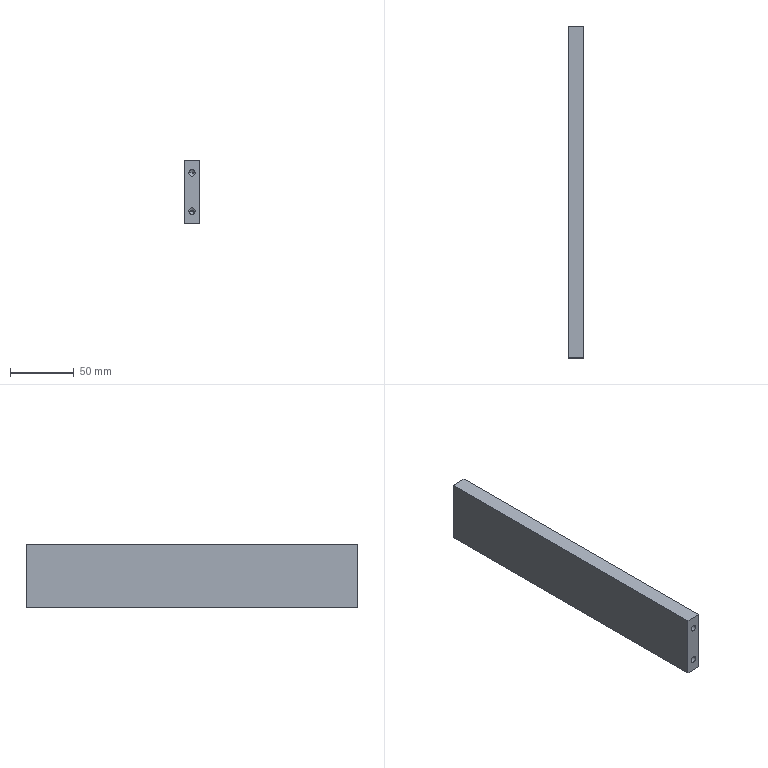Component | SolidWorks | AdjustmentSupportPlate-1 | 1 solid | 22 faces | box 12 x 260 x 50 mm | volume 154783 mm3 | cylinder 8 | cone 8 | plane 6 | commonest cylinder face diameters 5 x8
build123d program:
from build123d import *

# Parameters (mm, degrees)
SKETCH1_W             = 260
SKETCH1_H             = 50
EXTRUDE1_DEPTH        = 12
M6_TAPPED_HOLE1_D     = 5
M6_TAPPED_HOLE1_DEPTH = 15
M6_TAPPED_HOLE1_TIP   = 1.502
M6_TAPPED_HOLE2_D     = 5
M6_TAPPED_HOLE2_DEPTH = 15
M6_TAPPED_HOLE2_TIP   = 1.502


with BuildPart() as part:
    # Sketch1 → Extrude1 (new body)
    with BuildSketch(Plane.XY):
        with Locations((107.997, -15.106)):
            Rectangle(SKETCH1_W, SKETCH1_H)
    extrude(amount=EXTRUDE1_DEPTH)

    # M6 Tapped Hole1
    with Locations(Plane(origin=(237.997, -0.1058, 6), x_dir=(0, 1, 0), z_dir=(1, 0, 0))):
        with Locations((0, 0), (-30, 0)):
            Hole(M6_TAPPED_HOLE1_D / 2, depth=M6_TAPPED_HOLE1_DEPTH)
            with Locations((0, 0, -(M6_TAPPED_HOLE1_DEPTH + M6_TAPPED_HOLE1_TIP / 2))):  # 118° drill point
                Cone(0, M6_TAPPED_HOLE1_D / 2, M6_TAPPED_HOLE1_TIP, mode=Mode.SUBTRACT)

    # M6 Tapped Hole2
    with Locations(Plane(origin=(-22.003, -0.1058, 6), x_dir=(0, -1, 0), z_dir=(-1, 0, 0))):
        with Locations((0, 0), (30, 0)):
            Hole(M6_TAPPED_HOLE2_D / 2, depth=M6_TAPPED_HOLE2_DEPTH)
            with Locations((0, 0, -(M6_TAPPED_HOLE2_DEPTH + M6_TAPPED_HOLE2_TIP / 2))):  # 118° drill point
                Cone(0, M6_TAPPED_HOLE2_D / 2, M6_TAPPED_HOLE2_TIP, mode=Mode.SUBTRACT)


solid = part.part

# Placed as in the assembly
solid = solid.moved(Location((-285.284, 683.98, -65.394), (90, -90, 0)))
STEP:
#1=COLOUR_RGB('',0.7922,0.8196,0.9333);
#2=FILL_AREA_STYLE_COLOUR('',#1);
#3=FILL_AREA_STYLE('',(#2));
#4=SURFACE_STYLE_FILL_AREA(#3);
#5=SURFACE_SIDE_STYLE('',(#4));
#6=SURFACE_STYLE_USAGE(.BOTH.,#5);
#7=PRESENTATION_STYLE_ASSIGNMENT((#6));
#8=CARTESIAN_POINT('',(-11.566,27.204,-3.76));
#9=VERTEX_POINT('',#8);
#10=CARTESIAN_POINT('',(-11.369,27.204,-3.76));
#11=VERTEX_POINT('',#10);
#12=CARTESIAN_POINT('',(-11.468,27.204,-3.76));
#13=DIRECTION('',(-0.,1.,-0.));
#14=DIRECTION('',(1.,0.,-0.));
#15=AXIS2_PLACEMENT_3D('',#12,#13,#14);
#16=CIRCLE('',#15,0.09843);
#17=EDGE_CURVE('',#9,#11,#16,.T.);
#18=ORIENTED_EDGE('',*,*,#17,.F.);
#19=CARTESIAN_POINT('',(-11.566,27.795,-3.76));
#20=VERTEX_POINT('',#19);
#21=CARTESIAN_POINT('',(-11.566,27.795,-3.76));
#22=DIRECTION('',(-0.,1.,-0.));
#23=VECTOR('',#22,39.37);
#24=LINE('',#21,#23);
#25=EDGE_CURVE('',#9,#20,#24,.T.);
#26=ORIENTED_EDGE('',*,*,#25,.T.);
#27=CARTESIAN_POINT('',(-11.369,27.795,-3.76));
#28=VERTEX_POINT('',#27);
#29=CARTESIAN_POINT('',(-11.468,27.795,-3.76));
#30=DIRECTION('',(-0.,1.,-0.));
#31=DIRECTION('',(1.,0.,-0.));
#32=AXIS2_PLACEMENT_3D('',#29,#30,#31);
#33=CIRCLE('',#32,0.09843);
#34=EDGE_CURVE('',#20,#28,#33,.T.);
#35=ORIENTED_EDGE('',*,*,#34,.T.);
#36=CARTESIAN_POINT('',(-11.369,27.795,-3.76));
#37=DIRECTION('',(-0.,1.,-0.));
#38=VECTOR('',#37,39.37);
#39=LINE('',#36,#38);
#40=EDGE_CURVE('',#11,#28,#39,.T.);
#41=ORIENTED_EDGE('',*,*,#40,.F.);
#42=EDGE_LOOP('',(#18,#26,#35,#41));
#43=FACE_OUTER_BOUND('',#42,.T.);
#44=CARTESIAN_POINT('',(-11.468,27.795,-3.76));
#45=DIRECTION('',(-0.,1.,-0.));
#46=DIRECTION('',(1.,0.,-0.));
#47=AXIS2_PLACEMENT_3D('',#44,#45,#46);
#48=CYLINDRICAL_SURFACE('',#47,0.09843);
#49=ADVANCED_FACE('',(#43),#48,.F.);
#50=CARTESIAN_POINT('',(-11.468,27.145,-3.76));
#51=VERTEX_POINT('',#50);
#52=CARTESIAN_POINT('',(-11.369,27.204,-3.76));
#53=DIRECTION('',(0.8572,0.515,-0.));
#54=VECTOR('',#53,39.37);
#55=LINE('',#52,#54);
#56=EDGE_CURVE('',#51,#11,#55,.T.);
#57=ORIENTED_EDGE('',*,*,#56,.F.);
#58=CARTESIAN_POINT('',(-11.566,27.204,-3.76));
#59=DIRECTION('',(-0.8572,0.515,0.));
#60=VECTOR('',#59,39.37);
#61=LINE('',#58,#60);
#62=EDGE_CURVE('',#51,#9,#61,.T.);
#63=ORIENTED_EDGE('',*,*,#62,.T.);
#64=ORIENTED_EDGE('',*,*,#17,.T.);
#65=EDGE_LOOP('',(#57,#63,#64));
#66=FACE_OUTER_BOUND('',#65,.T.);
#67=CARTESIAN_POINT('',(-11.468,27.204,-3.76));
#68=DIRECTION('',(-0.,1.,-0.));
#69=DIRECTION('',(1.,0.,-0.));
#70=AXIS2_PLACEMENT_3D('',#67,#68,#69);
#71=CONICAL_SURFACE('',#70,0.09843,1.03);
#72=ADVANCED_FACE('',(#66),#71,.F.);
#73=CARTESIAN_POINT('',(-11.566,27.204,-2.579));
#74=VERTEX_POINT('',#73);
#75=CARTESIAN_POINT('',(-11.369,27.204,-2.579));
#76=VERTEX_POINT('',#75);
#77=CARTESIAN_POINT('',(-11.468,27.204,-2.579));
#78=DIRECTION('',(-0.,1.,-0.));
#79=DIRECTION('',(1.,0.,-0.));
#80=AXIS2_PLACEMENT_3D('',#77,#78,#79);
#81=CIRCLE('',#80,0.09843);
#82=EDGE_CURVE('',#74,#76,#81,.T.);
#83=ORIENTED_EDGE('',*,*,#82,.F.);
#84=CARTESIAN_POINT('',(-11.566,27.795,-2.579));
#85=VERTEX_POINT('',#84);
#86=CARTESIAN_POINT('',(-11.566,27.795,-2.579));
#87=DIRECTION('',(-0.,1.,-0.));
#88=VECTOR('',#87,39.37);
#89=LINE('',#86,#88);
#90=EDGE_CURVE('',#74,#85,#89,.T.);
#91=ORIENTED_EDGE('',*,*,#90,.T.);
#92=CARTESIAN_POINT('',(-11.369,27.795,-2.579));
#93=VERTEX_POINT('',#92);
#94=CARTESIAN_POINT('',(-11.468,27.795,-2.579));
#95=DIRECTION('',(-0.,1.,-0.));
#96=DIRECTION('',(1.,0.,-0.));
#97=AXIS2_PLACEMENT_3D('',#94,#95,#96);
#98=CIRCLE('',#97,0.09843);
#99=EDGE_CURVE('',#85,#93,#98,.T.);
#100=ORIENTED_EDGE('',*,*,#99,.T.);
#101=CARTESIAN_POINT('',(-11.369,27.795,-2.579));
#102=DIRECTION('',(-0.,1.,-0.));
#103=VECTOR('',#102,39.37);
#104=LINE('',#101,#103);
#105=EDGE_CURVE('',#76,#93,#104,.T.);
#106=ORIENTED_EDGE('',*,*,#105,.F.);
#107=EDGE_LOOP('',(#83,#91,#100,#106));
#108=FACE_OUTER_BOUND('',#107,.T.);
#109=CARTESIAN_POINT('',(-11.468,27.795,-2.579));
#110=DIRECTION('',(-0.,1.,-0.));
#111=DIRECTION('',(1.,0.,-0.));
#112=AXIS2_PLACEMENT_3D('',#109,#110,#111);
#113=CYLINDRICAL_SURFACE('',#112,0.09843);
#114=ADVANCED_FACE('',(#108),#113,.F.);
#115=CARTESIAN_POINT('',(-11.468,27.145,-2.579));
#116=VERTEX_POINT('',#115);
#117=CARTESIAN_POINT('',(-11.369,27.204,-2.579));
#118=DIRECTION('',(0.8572,0.515,-0.));
#119=VECTOR('',#118,39.37);
#120=LINE('',#117,#119);
#121=EDGE_CURVE('',#116,#76,#120,.T.);
#122=ORIENTED_EDGE('',*,*,#121,.F.);
#123=CARTESIAN_POINT('',(-11.566,27.204,-2.579));
#124=DIRECTION('',(-0.8572,0.515,0.));
#125=VECTOR('',#124,39.37);
#126=LINE('',#123,#125);
#127=EDGE_CURVE('',#116,#74,#126,.T.);
#128=ORIENTED_EDGE('',*,*,#127,.T.);
#129=ORIENTED_EDGE('',*,*,#82,.T.);
#130=EDGE_LOOP('',(#122,#128,#129));
#131=FACE_OUTER_BOUND('',#130,.T.);
#132=CARTESIAN_POINT('',(-11.468,27.204,-2.579));
#133=DIRECTION('',(-0.,1.,-0.));
#134=DIRECTION('',(1.,0.,-0.));
#135=AXIS2_PLACEMENT_3D('',#132,#133,#134);
#136=CONICAL_SURFACE('',#135,0.09843,1.03);
#137=ADVANCED_FACE('',(#131),#136,.F.);
#138=CARTESIAN_POINT('',(-11.369,18.149,-3.76));
#139=VERTEX_POINT('',#138);
#140=CARTESIAN_POINT('',(-11.566,18.149,-3.76));
#141=VERTEX_POINT('',#140);
#142=CARTESIAN_POINT('',(-11.468,18.149,-3.76));
#143=DIRECTION('',(0.,-1.,0.));
#144=DIRECTION('',(-1.,0.,0.));
#145=AXIS2_PLACEMENT_3D('',#142,#143,#144);
#146=CIRCLE('',#145,0.09843);
#147=EDGE_CURVE('',#139,#141,#146,.T.);
#148=ORIENTED_EDGE('',*,*,#147,.F.);
#149=CARTESIAN_POINT('',(-11.369,17.558,-3.76));
#150=VERTEX_POINT('',#149);
#151=CARTESIAN_POINT('',(-11.369,17.558,-3.76));
#152=DIRECTION('',(0.,-1.,0.));
#153=VECTOR('',#152,39.37);
#154=LINE('',#151,#153);
#155=EDGE_CURVE('',#139,#150,#154,.T.);
#156=ORIENTED_EDGE('',*,*,#155,.T.);
#157=CARTESIAN_POINT('',(-11.566,17.558,-3.76));
#158=VERTEX_POINT('',#157);
#159=CARTESIAN_POINT('',(-11.468,17.558,-3.76));
#160=DIRECTION('',(0.,-1.,0.));
#161=DIRECTION('',(-1.,0.,0.));
#162=AXIS2_PLACEMENT_3D('',#159,#160,#161);
#163=CIRCLE('',#162,0.09843);
#164=EDGE_CURVE('',#150,#158,#163,.T.);
#165=ORIENTED_EDGE('',*,*,#164,.T.);
#166=CARTESIAN_POINT('',(-11.566,17.558,-3.76));
#167=DIRECTION('',(0.,-1.,0.));
#168=VECTOR('',#167,39.37);
#169=LINE('',#166,#168);
#170=EDGE_CURVE('',#141,#158,#169,.T.);
#171=ORIENTED_EDGE('',*,*,#170,.F.);
#172=EDGE_LOOP('',(#148,#156,#165,#171));
#173=FACE_OUTER_BOUND('',#172,.T.);
#174=CARTESIAN_POINT('',(-11.468,17.558,-3.76));
#175=DIRECTION('',(0.,-1.,0.));
#176=DIRECTION('',(-1.,0.,0.));
#177=AXIS2_PLACEMENT_3D('',#174,#175,#176);
#178=CYLINDRICAL_SURFACE('',#177,0.09843);
#179=ADVANCED_FACE('',(#173),#178,.F.);
#180=CARTESIAN_POINT('',(-11.468,18.208,-3.76));
#181=VERTEX_POINT('',#180);
#182=CARTESIAN_POINT('',(-11.566,18.149,-3.76));
#183=DIRECTION('',(-0.8572,-0.515,0.));
#184=VECTOR('',#183,39.37);
#185=LINE('',#182,#184);
#186=EDGE_CURVE('',#181,#141,#185,.T.);
#187=ORIENTED_EDGE('',*,*,#186,.F.);
#188=CARTESIAN_POINT('',(-11.369,18.149,-3.76));
#189=DIRECTION('',(0.8572,-0.515,-0.));
#190=VECTOR('',#189,39.37);
#191=LINE('',#188,#190);
#192=EDGE_CURVE('',#181,#139,#191,.T.);
#193=ORIENTED_EDGE('',*,*,#192,.T.);
#194=ORIENTED_EDGE('',*,*,#147,.T.);
#195=EDGE_LOOP('',(#187,#193,#194));
#196=FACE_OUTER_BOUND('',#195,.T.);
#197=CARTESIAN_POINT('',(-11.468,18.149,-3.76));
#198=DIRECTION('',(0.,-1.,0.));
#199=DIRECTION('',(-1.,0.,0.));
#200=AXIS2_PLACEMENT_3D('',#197,#198,#199);
#201=CONICAL_SURFACE('',#200,0.09843,1.03);
#202=ADVANCED_FACE('',(#196),#201,.F.);
#203=CARTESIAN_POINT('',(-11.369,18.149,-2.579));
#204=VERTEX_POINT('',#203);
#205=CARTESIAN_POINT('',(-11.566,18.149,-2.579));
#206=VERTEX_POINT('',#205);
#207=CARTESIAN_POINT('',(-11.468,18.149,-2.579));
#208=DIRECTION('',(0.,-1.,0.));
#209=DIRECTION('',(-1.,0.,0.));
#210=AXIS2_PLACEMENT_3D('',#207,#208,#209);
#211=CIRCLE('',#210,0.09843);
#212=EDGE_CURVE('',#204,#206,#211,.T.);
#213=ORIENTED_EDGE('',*,*,#212,.F.);
#214=CARTESIAN_POINT('',(-11.369,17.558,-2.579));
#215=VERTEX_POINT('',#214);
#216=CARTESIAN_POINT('',(-11.369,17.558,-2.579));
#217=DIRECTION('',(0.,-1.,0.));
#218=VECTOR('',#217,39.37);
#219=LINE('',#216,#218);
#220=EDGE_CURVE('',#204,#215,#219,.T.);
#221=ORIENTED_EDGE('',*,*,#220,.T.);
#222=CARTESIAN_POINT('',(-11.566,17.558,-2.579));
#223=VERTEX_POINT('',#222);
#224=CARTESIAN_POINT('',(-11.468,17.558,-2.579));
#225=DIRECTION('',(0.,-1.,0.));
#226=DIRECTION('',(-1.,0.,0.));
#227=AXIS2_PLACEMENT_3D('',#224,#225,#226);
#228=CIRCLE('',#227,0.09843);
#229=EDGE_CURVE('',#215,#223,#228,.T.);
#230=ORIENTED_EDGE('',*,*,#229,.T.);
#231=CARTESIAN_POINT('',(-11.566,17.558,-2.579));
#232=DIRECTION('',(0.,-1.,0.));
#233=VECTOR('',#232,39.37);
#234=LINE('',#231,#233);
#235=EDGE_CURVE('',#206,#223,#234,.T.);
#236=ORIENTED_EDGE('',*,*,#235,.F.);
#237=EDGE_LOOP('',(#213,#221,#230,#236));
#238=FACE_OUTER_BOUND('',#237,.T.);
#239=CARTESIAN_POINT('',(-11.468,17.558,-2.579));
#240=DIRECTION('',(0.,-1.,0.));
#241=DIRECTION('',(-1.,0.,0.));
#242=AXIS2_PLACEMENT_3D('',#239,#240,#241);
#243=CYLINDRICAL_SURFACE('',#242,0.09843);
#244=ADVANCED_FACE('',(#238),#243,.F.);
#245=CARTESIAN_POINT('',(-11.468,18.208,-2.579));
#246=VERTEX_POINT('',#245);
#247=CARTESIAN_POINT('',(-11.566,18.149,-2.579));
#248=DIRECTION('',(-0.8572,-0.515,0.));
#249=VECTOR('',#248,39.37);
#250=LINE('',#247,#249);
#251=EDGE_CURVE('',#246,#206,#250,.T.);
#252=ORIENTED_EDGE('',*,*,#251,.F.);
#253=CARTESIAN_POINT('',(-11.369,18.149,-2.579));
#254=DIRECTION('',(0.8572,-0.515,-0.));
#255=VECTOR('',#254,39.37);
#256=LINE('',#253,#255);
#257=EDGE_CURVE('',#246,#204,#256,.T.);
#258=ORIENTED_EDGE('',*,*,#257,.T.);
#259=ORIENTED_EDGE('',*,*,#212,.T.);
#260=EDGE_LOOP('',(#252,#258,#259));
#261=FACE_OUTER_BOUND('',#260,.T.);
#262=CARTESIAN_POINT('',(-11.468,18.149,-2.579));
#263=DIRECTION('',(0.,-1.,0.));
#264=DIRECTION('',(-1.,0.,0.));
#265=AXIS2_PLACEMENT_3D('',#262,#263,#264);
#266=CONICAL_SURFACE('',#265,0.09843,1.03);
#267=ADVANCED_FACE('',(#261),#266,.F.);
#268=CARTESIAN_POINT('',(-11.468,27.795,-3.76));
#269=DIRECTION('',(-0.,1.,-0.));
#270=DIRECTION('',(1.,0.,-0.));
#271=AXIS2_PLACEMENT_3D('',#268,#269,#270);
#272=CIRCLE('',#271,0.09843);
#273=EDGE_CURVE('',#28,#20,#272,.T.);
#274=ORIENTED_EDGE('',*,*,#273,.F.);
#275=ORIENTED_EDGE('',*,*,#34,.F.);
#276=EDGE_LOOP('',(#274,#275));
#277=FACE_BOUND('',#276,.T.);
#278=CARTESIAN_POINT('',(-11.468,27.795,-2.579));
#279=DIRECTION('',(-0.,1.,-0.));
#280=DIRECTION('',(1.,0.,-0.));
#281=AXIS2_PLACEMENT_3D('',#278,#279,#280);
#282=CIRCLE('',#281,0.09843);
#283=EDGE_CURVE('',#93,#85,#282,.T.);
#284=ORIENTED_EDGE('',*,*,#283,.F.);
#285=ORIENTED_EDGE('',*,*,#99,.F.);
#286=EDGE_LOOP('',(#284,#285));
#287=FACE_BOUND('',#286,.T.);
#288=CARTESIAN_POINT('',(-11.704,27.795,-4.154));
#289=VERTEX_POINT('',#288);
#290=CARTESIAN_POINT('',(-11.704,27.795,-2.185));
#291=VERTEX_POINT('',#290);
#292=CARTESIAN_POINT('',(-11.704,27.795,-4.154));
#293=DIRECTION('',(0.,0.,1.));
#294=VECTOR('',#293,39.37);
#295=LINE('',#292,#294);
#296=EDGE_CURVE('',#289,#291,#295,.T.);
#297=ORIENTED_EDGE('',*,*,#296,.T.);
#298=CARTESIAN_POINT('',(-11.232,27.795,-2.185));
#299=VERTEX_POINT('',#298);
#300=CARTESIAN_POINT('',(-11.232,27.795,-2.185));
#301=DIRECTION('',(-1.,-0.,0.));
#302=VECTOR('',#301,39.37);
#303=LINE('',#300,#302);
#304=EDGE_CURVE('',#299,#291,#303,.T.);
#305=ORIENTED_EDGE('',*,*,#304,.F.);
#306=CARTESIAN_POINT('',(-11.232,27.795,-4.154));
#307=VERTEX_POINT('',#306);
#308=CARTESIAN_POINT('',(-11.232,27.795,-4.154));
#309=DIRECTION('',(0.,0.,1.));
#310=VECTOR('',#309,39.37);
#311=LINE('',#308,#310);
#312=EDGE_CURVE('',#307,#299,#311,.T.);
#313=ORIENTED_EDGE('',*,*,#312,.F.);
#314=CARTESIAN_POINT('',(-11.232,27.795,-4.154));
#315=DIRECTION('',(-1.,-0.,0.));
#316=VECTOR('',#315,39.37);
#317=LINE('',#314,#316);
#318=EDGE_CURVE('',#307,#289,#317,.T.);
#319=ORIENTED_EDGE('',*,*,#318,.T.);
#320=EDGE_LOOP('',(#297,#305,#313,#319));
#321=FACE_OUTER_BOUND('',#320,.T.);
#322=CARTESIAN_POINT('',(-11.232,27.795,-4.154));
#323=DIRECTION('',(0.,-1.,0.));
#324=DIRECTION('',(-0.,-0.,-1.));
#325=AXIS2_PLACEMENT_3D('',#322,#323,#324);
#326=PLANE('',#325);
#327=ADVANCED_FACE('',(#277,#287,#321),#326,.F.);
#328=CARTESIAN_POINT('',(-11.704,17.558,-2.185));
#329=VERTEX_POINT('',#328);
#330=CARTESIAN_POINT('',(-11.704,27.795,-2.185));
#331=DIRECTION('',(0.,-1.,0.));
#332=VECTOR('',#331,39.37);
#333=LINE('',#330,#332);
#334=EDGE_CURVE('',#291,#329,#333,.T.);
#335=ORIENTED_EDGE('',*,*,#334,.T.);
#336=CARTESIAN_POINT('',(-11.232,17.558,-2.185));
#337=VERTEX_POINT('',#336);
#338=CARTESIAN_POINT('',(-11.232,17.558,-2.185));
#339=DIRECTION('',(-1.,-0.,0.));
#340=VECTOR('',#339,39.37);
#341=LINE('',#338,#340);
#342=EDGE_CURVE('',#337,#329,#341,.T.);
#343=ORIENTED_EDGE('',*,*,#342,.F.);
#344=CARTESIAN_POINT('',(-11.232,27.795,-2.185));
#345=DIRECTION('',(0.,-1.,0.));
#346=VECTOR('',#345,39.37);
#347=LINE('',#344,#346);
#348=EDGE_CURVE('',#299,#337,#347,.T.);
#349=ORIENTED_EDGE('',*,*,#348,.F.);
#350=ORIENTED_EDGE('',*,*,#304,.T.);
#351=EDGE_LOOP('',(#335,#343,#349,#350));
#352=FACE_OUTER_BOUND('',#351,.T.);
#353=CARTESIAN_POINT('',(-11.232,27.795,-2.185));
#354=DIRECTION('',(-0.,-0.,-1.));
#355=DIRECTION('',(1.,0.,-0.));
#356=AXIS2_PLACEMENT_3D('',#353,#354,#355);
#357=PLANE('',#356);
#358=ADVANCED_FACE('',(#352),#357,.F.);
#359=CARTESIAN_POINT('',(-11.468,17.558,-3.76));
#360=DIRECTION('',(0.,-1.,0.));
#361=DIRECTION('',(-1.,0.,0.));
#362=AXIS2_PLACEMENT_3D('',#359,#360,#361);
#363=CIRCLE('',#362,0.09843);
#364=EDGE_CURVE('',#158,#150,#363,.T.);
#365=ORIENTED_EDGE('',*,*,#364,.F.);
#366=ORIENTED_EDGE('',*,*,#164,.F.);
#367=EDGE_LOOP('',(#365,#366));
#368=FACE_BOUND('',#367,.T.);
#369=CARTESIAN_POINT('',(-11.468,17.558,-2.579));
#370=DIRECTION('',(0.,-1.,0.));
#371=DIRECTION('',(-1.,0.,0.));
#372=AXIS2_PLACEMENT_3D('',#369,#370,#371);
#373=CIRCLE('',#372,0.09843);
#374=EDGE_CURVE('',#223,#215,#373,.T.);
#375=ORIENTED_EDGE('',*,*,#374,.F.);
#376=ORIENTED_EDGE('',*,*,#229,.F.);
#377=EDGE_LOOP('',(#375,#376));
#378=FACE_BOUND('',#377,.T.);
#379=CARTESIAN_POINT('',(-11.704,17.558,-4.154));
#380=VERTEX_POINT('',#379);
#381=CARTESIAN_POINT('',(-11.704,17.558,-4.154));
#382=DIRECTION('',(-0.,0.,-1.));
#383=VECTOR('',#382,39.37);
#384=LINE('',#381,#383);
#385=EDGE_CURVE('',#329,#380,#384,.T.);
#386=ORIENTED_EDGE('',*,*,#385,.T.);
#387=CARTESIAN_POINT('',(-11.232,17.558,-4.154));
#388=VERTEX_POINT('',#387);
#389=CARTESIAN_POINT('',(-11.232,17.558,-4.154));
#390=DIRECTION('',(-1.,-0.,0.));
#391=VECTOR('',#390,39.37);
#392=LINE('',#389,#391);
#393=EDGE_CURVE('',#388,#380,#392,.T.);
#394=ORIENTED_EDGE('',*,*,#393,.F.);
#395=CARTESIAN_POINT('',(-11.232,17.558,-4.154));
#396=DIRECTION('',(-0.,0.,-1.));
#397=VECTOR('',#396,39.37);
#398=LINE('',#395,#397);
#399=EDGE_CURVE('',#337,#388,#398,.T.);
#400=ORIENTED_EDGE('',*,*,#399,.F.);
#401=ORIENTED_EDGE('',*,*,#342,.T.);
#402=EDGE_LOOP('',(#386,#394,#400,#401));
#403=FACE_OUTER_BOUND('',#402,.T.);
#404=CARTESIAN_POINT('',(-11.232,17.558,-4.154));
#405=DIRECTION('',(-0.,1.,0.));
#406=DIRECTION('',(0.,-0.,1.));
#407=AXIS2_PLACEMENT_3D('',#404,#405,#406);
#408=PLANE('',#407);
#409=ADVANCED_FACE('',(#368,#378,#403),#408,.F.);
#410=CARTESIAN_POINT('',(-11.704,27.795,-4.154));
#411=DIRECTION('',(-0.,1.,-0.));
#412=VECTOR('',#411,39.37);
#413=LINE('',#410,#412);
#414=EDGE_CURVE('',#380,#289,#413,.T.);
#415=ORIENTED_EDGE('',*,*,#414,.T.);
#416=ORIENTED_EDGE('',*,*,#318,.F.);
#417=CARTESIAN_POINT('',(-11.232,27.795,-4.154));
#418=DIRECTION('',(-0.,1.,-0.));
#419=VECTOR('',#418,39.37);
#420=LINE('',#417,#419);
#421=EDGE_CURVE('',#388,#307,#420,.T.);
#422=ORIENTED_EDGE('',*,*,#421,.F.);
#423=ORIENTED_EDGE('',*,*,#393,.T.);
#424=EDGE_LOOP('',(#415,#416,#422,#423));
#425=FACE_OUTER_BOUND('',#424,.T.);
#426=CARTESIAN_POINT('',(-11.232,27.795,-4.154));
#427=DIRECTION('',(0.,0.,1.));
#428=DIRECTION('',(-1.,-0.,0.));
#429=AXIS2_PLACEMENT_3D('',#426,#427,#428);
#430=PLANE('',#429);
#431=ADVANCED_FACE('',(#425),#430,.F.);
#432=ORIENTED_EDGE('',*,*,#312,.T.);
#433=ORIENTED_EDGE('',*,*,#348,.T.);
#434=ORIENTED_EDGE('',*,*,#399,.T.);
#435=ORIENTED_EDGE('',*,*,#421,.T.);
#436=EDGE_LOOP('',(#432,#433,#434,#435));
#437=FACE_OUTER_BOUND('',#436,.T.);
#438=CARTESIAN_POINT('',(-11.232,27.795,-2.185));
#439=DIRECTION('',(1.,0.,-0.));
#440=DIRECTION('',(0.,-1.,0.));
#441=AXIS2_PLACEMENT_3D('',#438,#439,#440);
#442=PLANE('',#441);
#443=ADVANCED_FACE('',(#437),#442,.T.);
#444=ORIENTED_EDGE('',*,*,#296,.F.);
#445=ORIENTED_EDGE('',*,*,#414,.F.);
#446=ORIENTED_EDGE('',*,*,#385,.F.);
#447=ORIENTED_EDGE('',*,*,#334,.F.);
#448=EDGE_LOOP('',(#444,#445,#446,#447));
#449=FACE_OUTER_BOUND('',#448,.T.);
#450=CARTESIAN_POINT('',(-11.704,27.795,-2.185));
#451=DIRECTION('',(1.,0.,-0.));
#452=DIRECTION('',(0.,-1.,0.));
#453=AXIS2_PLACEMENT_3D('',#450,#451,#452);
#454=PLANE('',#453);
#455=ADVANCED_FACE('',(#449),#454,.F.);
#456=ORIENTED_EDGE('',*,*,#257,.F.);
#457=ORIENTED_EDGE('',*,*,#251,.T.);
#458=CARTESIAN_POINT('',(-11.468,18.149,-2.579));
#459=DIRECTION('',(0.,-1.,0.));
#460=DIRECTION('',(-1.,0.,0.));
#461=AXIS2_PLACEMENT_3D('',#458,#459,#460);
#462=CIRCLE('',#461,0.09843);
#463=EDGE_CURVE('',#206,#204,#462,.T.);
#464=ORIENTED_EDGE('',*,*,#463,.T.);
#465=EDGE_LOOP('',(#456,#457,#464));
#466=FACE_OUTER_BOUND('',#465,.T.);
#467=CARTESIAN_POINT('',(-11.468,18.149,-2.579));
#468=DIRECTION('',(0.,-1.,0.));
#469=DIRECTION('',(-1.,0.,0.));
#470=AXIS2_PLACEMENT_3D('',#467,#468,#469);
#471=CONICAL_SURFACE('',#470,0.09843,1.03);
#472=ADVANCED_FACE('',(#466),#471,.F.);
#473=ORIENTED_EDGE('',*,*,#220,.F.);
#474=ORIENTED_EDGE('',*,*,#463,.F.);
#475=ORIENTED_EDGE('',*,*,#235,.T.);
#476=ORIENTED_EDGE('',*,*,#374,.T.);
#477=EDGE_LOOP('',(#473,#474,#475,#476));
#478=FACE_OUTER_BOUND('',#477,.T.);
#479=CARTESIAN_POINT('',(-11.468,17.558,-2.579));
#480=DIRECTION('',(0.,-1.,0.));
#481=DIRECTION('',(-1.,0.,0.));
#482=AXIS2_PLACEMENT_3D('',#479,#480,#481);
#483=CYLINDRICAL_SURFACE('',#482,0.09843);
#484=ADVANCED_FACE('',(#478),#483,.F.);
#485=ORIENTED_EDGE('',*,*,#192,.F.);
#486=ORIENTED_EDGE('',*,*,#186,.T.);
#487=CARTESIAN_POINT('',(-11.468,18.149,-3.76));
#488=DIRECTION('',(0.,-1.,0.));
#489=DIRECTION('',(-1.,0.,0.));
#490=AXIS2_PLACEMENT_3D('',#487,#488,#489);
#491=CIRCLE('',#490,0.09843);
#492=EDGE_CURVE('',#141,#139,#491,.T.);
#493=ORIENTED_EDGE('',*,*,#492,.T.);
#494=EDGE_LOOP('',(#485,#486,#493));
#495=FACE_OUTER_BOUND('',#494,.T.);
#496=CARTESIAN_POINT('',(-11.468,18.149,-3.76));
#497=DIRECTION('',(0.,-1.,0.));
#498=DIRECTION('',(-1.,0.,0.));
#499=AXIS2_PLACEMENT_3D('',#496,#497,#498);
#500=CONICAL_SURFACE('',#499,0.09843,1.03);
#501=ADVANCED_FACE('',(#495),#500,.F.);
#502=ORIENTED_EDGE('',*,*,#155,.F.);
#503=ORIENTED_EDGE('',*,*,#492,.F.);
#504=ORIENTED_EDGE('',*,*,#170,.T.);
#505=ORIENTED_EDGE('',*,*,#364,.T.);
#506=EDGE_LOOP('',(#502,#503,#504,#505));
#507=FACE_OUTER_BOUND('',#506,.T.);
#508=CARTESIAN_POINT('',(-11.468,17.558,-3.76));
#509=DIRECTION('',(0.,-1.,0.));
#510=DIRECTION('',(-1.,0.,0.));
#511=AXIS2_PLACEMENT_3D('',#508,#509,#510);
#512=CYLINDRICAL_SURFACE('',#511,0.09843);
#513=ADVANCED_FACE('',(#507),#512,.F.);
#514=ORIENTED_EDGE('',*,*,#127,.F.);
#515=ORIENTED_EDGE('',*,*,#121,.T.);
#516=CARTESIAN_POINT('',(-11.468,27.204,-2.579));
#517=DIRECTION('',(-0.,1.,-0.));
#518=DIRECTION('',(1.,0.,-0.));
#519=AXIS2_PLACEMENT_3D('',#516,#517,#518);
#520=CIRCLE('',#519,0.09843);
#521=EDGE_CURVE('',#76,#74,#520,.T.);
#522=ORIENTED_EDGE('',*,*,#521,.T.);
#523=EDGE_LOOP('',(#514,#515,#522));
#524=FACE_OUTER_BOUND('',#523,.T.);
#525=CARTESIAN_POINT('',(-11.468,27.204,-2.579));
#526=DIRECTION('',(-0.,1.,-0.));
#527=DIRECTION('',(1.,0.,-0.));
#528=AXIS2_PLACEMENT_3D('',#525,#526,#527);
#529=CONICAL_SURFACE('',#528,0.09843,1.03);
#530=ADVANCED_FACE('',(#524),#529,.F.);
#531=ORIENTED_EDGE('',*,*,#90,.F.);
#532=ORIENTED_EDGE('',*,*,#521,.F.);
#533=ORIENTED_EDGE('',*,*,#105,.T.);
#534=ORIENTED_EDGE('',*,*,#283,.T.);
#535=EDGE_LOOP('',(#531,#532,#533,#534));
#536=FACE_OUTER_BOUND('',#535,.T.);
#537=CARTESIAN_POINT('',(-11.468,27.795,-2.579));
#538=DIRECTION('',(-0.,1.,-0.));
#539=DIRECTION('',(1.,0.,-0.));
#540=AXIS2_PLACEMENT_3D('',#537,#538,#539);
#541=CYLINDRICAL_SURFACE('',#540,0.09843);
#542=ADVANCED_FACE('',(#536),#541,.F.);
#543=ORIENTED_EDGE('',*,*,#62,.F.);
#544=ORIENTED_EDGE('',*,*,#56,.T.);
#545=CARTESIAN_POINT('',(-11.468,27.204,-3.76));
#546=DIRECTION('',(-0.,1.,-0.));
#547=DIRECTION('',(1.,0.,-0.));
#548=AXIS2_PLACEMENT_3D('',#545,#546,#547);
#549=CIRCLE('',#548,0.09843);
#550=EDGE_CURVE('',#11,#9,#549,.T.);
#551=ORIENTED_EDGE('',*,*,#550,.T.);
#552=EDGE_LOOP('',(#543,#544,#551));
#553=FACE_OUTER_BOUND('',#552,.T.);
#554=CARTESIAN_POINT('',(-11.468,27.204,-3.76));
#555=DIRECTION('',(-0.,1.,-0.));
#556=DIRECTION('',(1.,0.,-0.));
#557=AXIS2_PLACEMENT_3D('',#554,#555,#556);
#558=CONICAL_SURFACE('',#557,0.09843,1.03);
#559=ADVANCED_FACE('',(#553),#558,.F.);
#560=ORIENTED_EDGE('',*,*,#25,.F.);
#561=ORIENTED_EDGE('',*,*,#550,.F.);
#562=ORIENTED_EDGE('',*,*,#40,.T.);
#563=ORIENTED_EDGE('',*,*,#273,.T.);
#564=EDGE_LOOP('',(#560,#561,#562,#563));
#565=FACE_OUTER_BOUND('',#564,.T.);
#566=CARTESIAN_POINT('',(-11.468,27.795,-3.76));
#567=DIRECTION('',(-0.,1.,-0.));
#568=DIRECTION('',(1.,0.,-0.));
#569=AXIS2_PLACEMENT_3D('',#566,#567,#568);
#570=CYLINDRICAL_SURFACE('',#569,0.09843);
#571=ADVANCED_FACE('',(#565),#570,.F.);
#572=CLOSED_SHELL('',(#49,#72,#114,#137,#179,#202,#244,#267,#327,#358,#409,#431,#443,#455,#472,#484,#501,#513,#530,#542,#559,#571));
#573=MANIFOLD_SOLID_BREP('',#572);
#574=STYLED_ITEM('',(#7),#573);
#575=(LENGTH_UNIT()NAMED_UNIT(*)SI_UNIT($,.METRE.));
#576=LENGTH_MEASURE_WITH_UNIT(LENGTH_MEASURE(0.0254),#575);
#577=DIMENSIONAL_EXPONENTS(1.,0.,0.,0.,0.,0.,0.);
#578=(CONVERSION_BASED_UNIT('',#576)LENGTH_UNIT()NAMED_UNIT(#577));
#579=UNCERTAINTY_MEASURE_WITH_UNIT(LENGTH_MEASURE(0.00001),#578,'','');
#580=(NAMED_UNIT(*)PLANE_ANGLE_UNIT()SI_UNIT($,.RADIAN.));
#581=(NAMED_UNIT(*)SI_UNIT($,.STERADIAN.)SOLID_ANGLE_UNIT());
#582=(GEOMETRIC_REPRESENTATION_CONTEXT(3)GLOBAL_UNCERTAINTY_ASSIGNED_CONTEXT((#579))GLOBAL_UNIT_ASSIGNED_CONTEXT((#578,#580,#581))REPRESENTATION_CONTEXT('',''));
#583=MECHANICAL_DESIGN_GEOMETRIC_PRESENTATION_REPRESENTATION('',(#574),#582);
#584=CARTESIAN_POINT('',(0.,0.,0.));
#585=DIRECTION('',(0.,0.,1.));
#586=DIRECTION('',(1.,0.,0.));
#587=AXIS2_PLACEMENT_3D('',#584,#585,#586);
#588=(LENGTH_UNIT()NAMED_UNIT(*)SI_UNIT($,.METRE.));
#589=LENGTH_MEASURE_WITH_UNIT(LENGTH_MEASURE(0.0254),#588);
#590=DIMENSIONAL_EXPONENTS(1.,0.,0.,0.,0.,0.,0.);
#591=(CONVERSION_BASED_UNIT('',#589)LENGTH_UNIT()NAMED_UNIT(#590));
#592=UNCERTAINTY_MEASURE_WITH_UNIT(LENGTH_MEASURE(0.00001),#591,'','');
#593=(NAMED_UNIT(*)PLANE_ANGLE_UNIT()SI_UNIT($,.RADIAN.));
#594=(NAMED_UNIT(*)SI_UNIT($,.STERADIAN.)SOLID_ANGLE_UNIT());
#595=(GEOMETRIC_REPRESENTATION_CONTEXT(3)GLOBAL_UNCERTAINTY_ASSIGNED_CONTEXT((#592))GLOBAL_UNIT_ASSIGNED_CONTEXT((#591,#593,#594))REPRESENTATION_CONTEXT('',''));
#596=ADVANCED_BREP_SHAPE_REPRESENTATION('',(#573,#587),#595);
#597=PRESENTATION_LAYER_ASSIGNMENT('','',(#574));